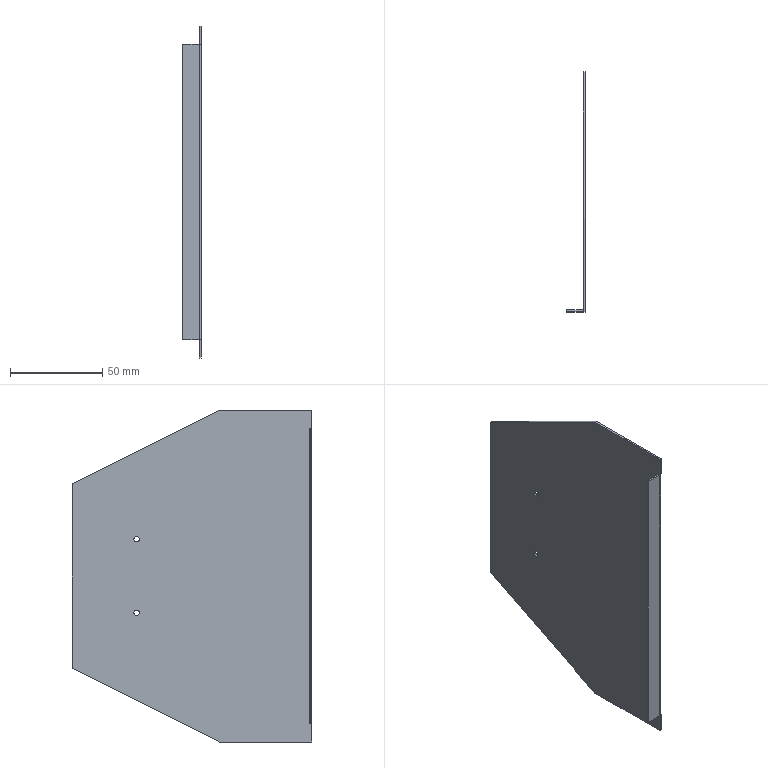Component | SolidWorks | LightBox-1_LightBox2-1 | 1 solid | 24 faces | box 10 x 130 x 180 mm | volume 21585 mm3 | plane 18 | cylinder 6 | commonest cylinder face diameters 3 x4 2.2 x1 0.2 x1
STEP:
#1=CARTESIAN_POINT('',(5.006,-0.2003,2.421));
#2=VERTEX_POINT('',#1);
#3=CARTESIAN_POINT('',(5.006,-0.2003,2.303));
#4=VERTEX_POINT('',#3);
#5=CARTESIAN_POINT('',(5.006,-0.2003,2.362));
#6=DIRECTION('',(1.,0.,0.));
#7=DIRECTION('',(0.,0.,-1.));
#8=AXIS2_PLACEMENT_3D('',#5,#6,#7);
#9=CIRCLE('',#8,0.05906);
#10=EDGE_CURVE('',#2,#4,#9,.T.);
#11=ORIENTED_EDGE('',*,*,#10,.F.);
#12=CARTESIAN_POINT('',(5.045,-0.2003,2.421));
#13=VERTEX_POINT('',#12);
#14=CARTESIAN_POINT('',(5.006,-0.2003,2.421));
#15=DIRECTION('',(1.,0.,0.));
#16=VECTOR('',#15,39.37);
#17=LINE('',#14,#16);
#18=EDGE_CURVE('',#2,#13,#17,.T.);
#19=ORIENTED_EDGE('',*,*,#18,.T.);
#20=CARTESIAN_POINT('',(5.045,-0.2003,2.303));
#21=VERTEX_POINT('',#20);
#22=CARTESIAN_POINT('',(5.045,-0.2003,2.362));
#23=DIRECTION('',(1.,0.,0.));
#24=DIRECTION('',(0.,0.,-1.));
#25=AXIS2_PLACEMENT_3D('',#22,#23,#24);
#26=CIRCLE('',#25,0.05906);
#27=EDGE_CURVE('',#13,#21,#26,.T.);
#28=ORIENTED_EDGE('',*,*,#27,.T.);
#29=CARTESIAN_POINT('',(5.006,-0.2003,2.303));
#30=DIRECTION('',(1.,0.,0.));
#31=VECTOR('',#30,39.37);
#32=LINE('',#29,#31);
#33=EDGE_CURVE('',#4,#21,#32,.T.);
#34=ORIENTED_EDGE('',*,*,#33,.F.);
#35=EDGE_LOOP('',(#11,#19,#28,#34));
#36=FACE_OUTER_BOUND('',#35,.T.);
#37=CARTESIAN_POINT('',(5.006,-0.2003,2.362));
#38=DIRECTION('',(1.,0.,0.));
#39=DIRECTION('',(0.,0.,-1.));
#40=AXIS2_PLACEMENT_3D('',#37,#38,#39);
#41=CYLINDRICAL_SURFACE('',#40,0.05906);
#42=ADVANCED_FACE('',(#36),#41,.F.);
#43=CARTESIAN_POINT('',(5.006,-0.2003,3.996));
#44=VERTEX_POINT('',#43);
#45=CARTESIAN_POINT('',(5.006,-0.2003,3.878));
#46=VERTEX_POINT('',#45);
#47=CARTESIAN_POINT('',(5.006,-0.2003,3.937));
#48=DIRECTION('',(1.,0.,0.));
#49=DIRECTION('',(0.,0.,-1.));
#50=AXIS2_PLACEMENT_3D('',#47,#48,#49);
#51=CIRCLE('',#50,0.05906);
#52=EDGE_CURVE('',#44,#46,#51,.T.);
#53=ORIENTED_EDGE('',*,*,#52,.F.);
#54=CARTESIAN_POINT('',(5.045,-0.2003,3.996));
#55=VERTEX_POINT('',#54);
#56=CARTESIAN_POINT('',(5.006,-0.2003,3.996));
#57=DIRECTION('',(1.,0.,0.));
#58=VECTOR('',#57,39.37);
#59=LINE('',#56,#58);
#60=EDGE_CURVE('',#44,#55,#59,.T.);
#61=ORIENTED_EDGE('',*,*,#60,.T.);
#62=CARTESIAN_POINT('',(5.045,-0.2003,3.878));
#63=VERTEX_POINT('',#62);
#64=CARTESIAN_POINT('',(5.045,-0.2003,3.937));
#65=DIRECTION('',(1.,0.,0.));
#66=DIRECTION('',(0.,0.,-1.));
#67=AXIS2_PLACEMENT_3D('',#64,#65,#66);
#68=CIRCLE('',#67,0.05906);
#69=EDGE_CURVE('',#55,#63,#68,.T.);
#70=ORIENTED_EDGE('',*,*,#69,.T.);
#71=CARTESIAN_POINT('',(5.006,-0.2003,3.878));
#72=DIRECTION('',(1.,0.,0.));
#73=VECTOR('',#72,39.37);
#74=LINE('',#71,#73);
#75=EDGE_CURVE('',#46,#63,#74,.T.);
#76=ORIENTED_EDGE('',*,*,#75,.F.);
#77=EDGE_LOOP('',(#53,#61,#70,#76));
#78=FACE_OUTER_BOUND('',#77,.T.);
#79=CARTESIAN_POINT('',(5.006,-0.2003,3.937));
#80=DIRECTION('',(1.,0.,0.));
#81=DIRECTION('',(0.,0.,-1.));
#82=AXIS2_PLACEMENT_3D('',#79,#80,#81);
#83=CYLINDRICAL_SURFACE('',#82,0.05906);
#84=ADVANCED_FACE('',(#78),#83,.F.);
#85=CARTESIAN_POINT('',(5.006,-3.94,6.299));
#86=VERTEX_POINT('',#85);
#87=CARTESIAN_POINT('',(5.006,-3.94,6.299));
#88=VERTEX_POINT('',#87);
#89=CARTESIAN_POINT('',(5.006,-3.94,6.299));
#90=DIRECTION('',(0.,1.,0.));
#91=VECTOR('',#90,39.37);
#92=LINE('',#89,#91);
#93=EDGE_CURVE('',#86,#88,#92,.T.);
#94=ORIENTED_EDGE('',*,*,#93,.T.);
#95=CARTESIAN_POINT('',(5.045,-3.897,6.299));
#96=VERTEX_POINT('',#95);
#97=CARTESIAN_POINT('',(5.002,-3.897,6.299));
#98=DIRECTION('',(0.,0.,1.));
#99=DIRECTION('',(1.,0.,0.));
#100=AXIS2_PLACEMENT_3D('',#97,#98,#99);
#101=CIRCLE('',#100,0.04331);
#102=EDGE_CURVE('',#88,#96,#101,.T.);
#103=ORIENTED_EDGE('',*,*,#102,.T.);
#104=CARTESIAN_POINT('',(5.045,-3.94,6.299));
#105=VERTEX_POINT('',#104);
#106=CARTESIAN_POINT('',(5.045,-0.9737,6.299));
#107=DIRECTION('',(0.,-1.,0.));
#108=VECTOR('',#107,39.37);
#109=LINE('',#106,#108);
#110=EDGE_CURVE('',#96,#105,#109,.T.);
#111=ORIENTED_EDGE('',*,*,#110,.T.);
#112=CARTESIAN_POINT('',(5.006,-3.94,6.299));
#113=DIRECTION('',(1.,0.,0.));
#114=VECTOR('',#113,39.37);
#115=LINE('',#112,#114);
#116=EDGE_CURVE('',#86,#105,#115,.T.);
#117=ORIENTED_EDGE('',*,*,#116,.F.);
#118=EDGE_LOOP('',(#94,#103,#111,#117));
#119=FACE_OUTER_BOUND('',#118,.T.);
#120=CARTESIAN_POINT('',(5.006,-3.94,6.299));
#121=DIRECTION('',(0.,-0.,-1.));
#122=DIRECTION('',(-1.,0.,-0.));
#123=AXIS2_PLACEMENT_3D('',#120,#121,#122);
#124=PLANE('',#123);
#125=ADVANCED_FACE('',(#119),#124,.T.);
#126=CARTESIAN_POINT('',(5.045,-3.94,0.));
#127=VERTEX_POINT('',#126);
#128=CARTESIAN_POINT('',(5.045,-3.897,0.));
#129=VERTEX_POINT('',#128);
#130=CARTESIAN_POINT('',(5.045,-0.9737,0.));
#131=DIRECTION('',(0.,1.,0.));
#132=VECTOR('',#131,39.37);
#133=LINE('',#130,#132);
#134=EDGE_CURVE('',#127,#129,#133,.T.);
#135=ORIENTED_EDGE('',*,*,#134,.T.);
#136=CARTESIAN_POINT('',(5.006,-3.94,0.));
#137=VERTEX_POINT('',#136);
#138=CARTESIAN_POINT('',(5.002,-3.897,0.));
#139=DIRECTION('',(-0.,0.,-1.));
#140=DIRECTION('',(1.,0.,-0.));
#141=AXIS2_PLACEMENT_3D('',#138,#139,#140);
#142=CIRCLE('',#141,0.04331);
#143=EDGE_CURVE('',#129,#137,#142,.T.);
#144=ORIENTED_EDGE('',*,*,#143,.T.);
#145=CARTESIAN_POINT('',(5.006,-3.94,0.));
#146=VERTEX_POINT('',#145);
#147=CARTESIAN_POINT('',(5.006,-3.897,0.));
#148=DIRECTION('',(0.,-1.,0.));
#149=VECTOR('',#148,39.37);
#150=LINE('',#147,#149);
#151=EDGE_CURVE('',#137,#146,#150,.T.);
#152=ORIENTED_EDGE('',*,*,#151,.T.);
#153=CARTESIAN_POINT('',(5.006,-3.94,0.));
#154=DIRECTION('',(1.,0.,0.));
#155=VECTOR('',#154,39.37);
#156=LINE('',#153,#155);
#157=EDGE_CURVE('',#146,#127,#156,.T.);
#158=ORIENTED_EDGE('',*,*,#157,.T.);
#159=EDGE_LOOP('',(#135,#144,#152,#158));
#160=FACE_OUTER_BOUND('',#159,.T.);
#161=CARTESIAN_POINT('',(5.006,-3.897,0.));
#162=DIRECTION('',(-0.,-0.,1.));
#163=DIRECTION('',(1.,0.,0.));
#164=AXIS2_PLACEMENT_3D('',#161,#162,#163);
#165=PLANE('',#164);
#166=ADVANCED_FACE('',(#160),#165,.T.);
#167=CARTESIAN_POINT('',(5.006,-3.94,6.693));
#168=VERTEX_POINT('',#167);
#169=CARTESIAN_POINT('',(5.006,-3.94,-0.3937));
#170=DIRECTION('',(0.,0.,-1.));
#171=VECTOR('',#170,39.37);
#172=LINE('',#169,#171);
#173=EDGE_CURVE('',#168,#86,#172,.T.);
#174=ORIENTED_EDGE('',*,*,#173,.T.);
#175=ORIENTED_EDGE('',*,*,#116,.T.);
#176=CARTESIAN_POINT('',(5.045,-3.94,6.693));
#177=VERTEX_POINT('',#176);
#178=CARTESIAN_POINT('',(5.045,-3.94,-0.3937));
#179=DIRECTION('',(0.,0.,-1.));
#180=VECTOR('',#179,39.37);
#181=LINE('',#178,#180);
#182=EDGE_CURVE('',#177,#105,#181,.T.);
#183=ORIENTED_EDGE('',*,*,#182,.F.);
#184=CARTESIAN_POINT('',(5.006,-3.94,6.693));
#185=DIRECTION('',(1.,0.,0.));
#186=VECTOR('',#185,39.37);
#187=LINE('',#184,#186);
#188=EDGE_CURVE('',#168,#177,#187,.T.);
#189=ORIENTED_EDGE('',*,*,#188,.F.);
#190=EDGE_LOOP('',(#174,#175,#183,#189));
#191=FACE_OUTER_BOUND('',#190,.T.);
#192=CARTESIAN_POINT('',(5.006,-3.94,-0.3937));
#193=DIRECTION('',(0.,-1.,-0.));
#194=DIRECTION('',(0.,0.,-1.));
#195=AXIS2_PLACEMENT_3D('',#192,#193,#194);
#196=PLANE('',#195);
#197=ADVANCED_FACE('',(#191),#196,.T.);
#198=CARTESIAN_POINT('',(5.045,-3.94,-0.3937));
#199=VERTEX_POINT('',#198);
#200=CARTESIAN_POINT('',(5.045,-3.94,-0.3937));
#201=DIRECTION('',(0.,0.,-1.));
#202=VECTOR('',#201,39.37);
#203=LINE('',#200,#202);
#204=EDGE_CURVE('',#127,#199,#203,.T.);
#205=ORIENTED_EDGE('',*,*,#204,.F.);
#206=ORIENTED_EDGE('',*,*,#157,.F.);
#207=CARTESIAN_POINT('',(5.006,-3.94,-0.3937));
#208=VERTEX_POINT('',#207);
#209=CARTESIAN_POINT('',(5.006,-3.94,-0.3937));
#210=DIRECTION('',(0.,0.,-1.));
#211=VECTOR('',#210,39.37);
#212=LINE('',#209,#211);
#213=EDGE_CURVE('',#146,#208,#212,.T.);
#214=ORIENTED_EDGE('',*,*,#213,.T.);
#215=CARTESIAN_POINT('',(5.006,-3.94,-0.3937));
#216=DIRECTION('',(1.,0.,0.));
#217=VECTOR('',#216,39.37);
#218=LINE('',#215,#217);
#219=EDGE_CURVE('',#208,#199,#218,.T.);
#220=ORIENTED_EDGE('',*,*,#219,.T.);
#221=EDGE_LOOP('',(#205,#206,#214,#220));
#222=FACE_OUTER_BOUND('',#221,.T.);
#223=CARTESIAN_POINT('',(5.006,-3.94,-0.3937));
#224=DIRECTION('',(0.,-1.,-0.));
#225=DIRECTION('',(0.,0.,-1.));
#226=AXIS2_PLACEMENT_3D('',#223,#224,#225);
#227=PLANE('',#226);
#228=ADVANCED_FACE('',(#222),#227,.T.);
#229=CARTESIAN_POINT('',(5.006,-0.2003,2.362));
#230=DIRECTION('',(1.,0.,0.));
#231=DIRECTION('',(0.,0.,-1.));
#232=AXIS2_PLACEMENT_3D('',#229,#230,#231);
#233=CIRCLE('',#232,0.05906);
#234=EDGE_CURVE('',#4,#2,#233,.T.);
#235=ORIENTED_EDGE('',*,*,#234,.T.);
#236=ORIENTED_EDGE('',*,*,#10,.T.);
#237=EDGE_LOOP('',(#235,#236));
#238=FACE_BOUND('',#237,.T.);
#239=CARTESIAN_POINT('',(5.006,-0.2003,3.937));
#240=DIRECTION('',(1.,0.,0.));
#241=DIRECTION('',(0.,0.,-1.));
#242=AXIS2_PLACEMENT_3D('',#239,#240,#241);
#243=CIRCLE('',#242,0.05906);
#244=EDGE_CURVE('',#46,#44,#243,.T.);
#245=ORIENTED_EDGE('',*,*,#244,.T.);
#246=ORIENTED_EDGE('',*,*,#52,.T.);
#247=EDGE_LOOP('',(#245,#246));
#248=FACE_BOUND('',#247,.T.);
#249=CARTESIAN_POINT('',(5.006,-3.897,6.299));
#250=VERTEX_POINT('',#249);
#251=CARTESIAN_POINT('',(5.006,-3.897,0.));
#252=VERTEX_POINT('',#251);
#253=CARTESIAN_POINT('',(5.006,-3.897,6.299));
#254=DIRECTION('',(-0.,0.,-1.));
#255=VECTOR('',#254,39.37);
#256=LINE('',#253,#255);
#257=EDGE_CURVE('',#250,#252,#256,.T.);
#258=ORIENTED_EDGE('',*,*,#257,.F.);
#259=CARTESIAN_POINT('',(5.006,-3.94,6.299));
#260=DIRECTION('',(0.,1.,0.));
#261=VECTOR('',#260,39.37);
#262=LINE('',#259,#261);
#263=EDGE_CURVE('',#88,#250,#262,.T.);
#264=ORIENTED_EDGE('',*,*,#263,.F.);
#265=ORIENTED_EDGE('',*,*,#93,.F.);
#266=ORIENTED_EDGE('',*,*,#173,.F.);
#267=CARTESIAN_POINT('',(5.006,-1.972,6.693));
#268=VERTEX_POINT('',#267);
#269=CARTESIAN_POINT('',(5.006,-3.94,6.693));
#270=DIRECTION('',(0.,-1.,0.));
#271=VECTOR('',#270,39.37);
#272=LINE('',#269,#271);
#273=EDGE_CURVE('',#268,#168,#272,.T.);
#274=ORIENTED_EDGE('',*,*,#273,.F.);
#275=CARTESIAN_POINT('',(5.006,1.178,5.118));
#276=VERTEX_POINT('',#275);
#277=CARTESIAN_POINT('',(5.006,-1.972,6.693));
#278=DIRECTION('',(0.,-0.8944,0.4472));
#279=VECTOR('',#278,39.37);
#280=LINE('',#277,#279);
#281=EDGE_CURVE('',#276,#268,#280,.T.);
#282=ORIENTED_EDGE('',*,*,#281,.F.);
#283=CARTESIAN_POINT('',(5.006,1.178,1.181));
#284=VERTEX_POINT('',#283);
#285=CARTESIAN_POINT('',(5.006,1.178,5.118));
#286=DIRECTION('',(0.,0.,1.));
#287=VECTOR('',#286,39.37);
#288=LINE('',#285,#287);
#289=EDGE_CURVE('',#284,#276,#288,.T.);
#290=ORIENTED_EDGE('',*,*,#289,.F.);
#291=CARTESIAN_POINT('',(5.006,-1.972,-0.3937));
#292=VERTEX_POINT('',#291);
#293=CARTESIAN_POINT('',(5.006,1.178,1.181));
#294=DIRECTION('',(0.,0.8944,0.4472));
#295=VECTOR('',#294,39.37);
#296=LINE('',#293,#295);
#297=EDGE_CURVE('',#292,#284,#296,.T.);
#298=ORIENTED_EDGE('',*,*,#297,.F.);
#299=CARTESIAN_POINT('',(5.006,-1.972,-0.3937));
#300=DIRECTION('',(0.,1.,0.));
#301=VECTOR('',#300,39.37);
#302=LINE('',#299,#301);
#303=EDGE_CURVE('',#208,#292,#302,.T.);
#304=ORIENTED_EDGE('',*,*,#303,.F.);
#305=ORIENTED_EDGE('',*,*,#213,.F.);
#306=ORIENTED_EDGE('',*,*,#151,.F.);
#307=CARTESIAN_POINT('',(5.006,-3.897,0.));
#308=DIRECTION('',(0.,-1.,0.));
#309=VECTOR('',#308,39.37);
#310=LINE('',#307,#309);
#311=EDGE_CURVE('',#252,#137,#310,.T.);
#312=ORIENTED_EDGE('',*,*,#311,.F.);
#313=EDGE_LOOP('',(#258,#264,#265,#266,#274,#282,#290,#298,#304,#305,#306,#312));
#314=FACE_OUTER_BOUND('',#313,.T.);
#315=CARTESIAN_POINT('',(5.006,-0.9737,3.033));
#316=DIRECTION('',(-1.,0.,0.));
#317=DIRECTION('',(0.,0.,1.));
#318=AXIS2_PLACEMENT_3D('',#315,#316,#317);
#319=PLANE('',#318);
#320=ADVANCED_FACE('',(#238,#248,#314),#319,.T.);
#321=CARTESIAN_POINT('',(5.045,-0.2003,3.937));
#322=DIRECTION('',(1.,0.,0.));
#323=DIRECTION('',(0.,0.,-1.));
#324=AXIS2_PLACEMENT_3D('',#321,#322,#323);
#325=CIRCLE('',#324,0.05906);
#326=EDGE_CURVE('',#63,#55,#325,.T.);
#327=ORIENTED_EDGE('',*,*,#326,.F.);
#328=ORIENTED_EDGE('',*,*,#69,.F.);
#329=EDGE_LOOP('',(#327,#328));
#330=FACE_BOUND('',#329,.T.);
#331=CARTESIAN_POINT('',(5.045,-0.2003,2.362));
#332=DIRECTION('',(1.,0.,0.));
#333=DIRECTION('',(0.,0.,-1.));
#334=AXIS2_PLACEMENT_3D('',#331,#332,#333);
#335=CIRCLE('',#334,0.05906);
#336=EDGE_CURVE('',#21,#13,#335,.T.);
#337=ORIENTED_EDGE('',*,*,#336,.F.);
#338=ORIENTED_EDGE('',*,*,#27,.F.);
#339=EDGE_LOOP('',(#337,#338));
#340=FACE_BOUND('',#339,.T.);
#341=ORIENTED_EDGE('',*,*,#110,.F.);
#342=CARTESIAN_POINT('',(5.045,-3.897,6.299));
#343=DIRECTION('',(-0.,0.,-1.));
#344=VECTOR('',#343,39.37);
#345=LINE('',#342,#344);
#346=EDGE_CURVE('',#96,#129,#345,.T.);
#347=ORIENTED_EDGE('',*,*,#346,.T.);
#348=ORIENTED_EDGE('',*,*,#134,.F.);
#349=ORIENTED_EDGE('',*,*,#204,.T.);
#350=CARTESIAN_POINT('',(5.045,-1.972,-0.3937));
#351=VERTEX_POINT('',#350);
#352=CARTESIAN_POINT('',(5.045,-1.972,-0.3937));
#353=DIRECTION('',(0.,1.,0.));
#354=VECTOR('',#353,39.37);
#355=LINE('',#352,#354);
#356=EDGE_CURVE('',#199,#351,#355,.T.);
#357=ORIENTED_EDGE('',*,*,#356,.T.);
#358=CARTESIAN_POINT('',(5.045,1.178,1.181));
#359=VERTEX_POINT('',#358);
#360=CARTESIAN_POINT('',(5.045,1.178,1.181));
#361=DIRECTION('',(0.,0.8944,0.4472));
#362=VECTOR('',#361,39.37);
#363=LINE('',#360,#362);
#364=EDGE_CURVE('',#351,#359,#363,.T.);
#365=ORIENTED_EDGE('',*,*,#364,.T.);
#366=CARTESIAN_POINT('',(5.045,1.178,5.118));
#367=VERTEX_POINT('',#366);
#368=CARTESIAN_POINT('',(5.045,1.178,5.118));
#369=DIRECTION('',(0.,0.,1.));
#370=VECTOR('',#369,39.37);
#371=LINE('',#368,#370);
#372=EDGE_CURVE('',#359,#367,#371,.T.);
#373=ORIENTED_EDGE('',*,*,#372,.T.);
#374=CARTESIAN_POINT('',(5.045,-1.972,6.693));
#375=VERTEX_POINT('',#374);
#376=CARTESIAN_POINT('',(5.045,-1.972,6.693));
#377=DIRECTION('',(0.,-0.8944,0.4472));
#378=VECTOR('',#377,39.37);
#379=LINE('',#376,#378);
#380=EDGE_CURVE('',#367,#375,#379,.T.);
#381=ORIENTED_EDGE('',*,*,#380,.T.);
#382=CARTESIAN_POINT('',(5.045,-3.94,6.693));
#383=DIRECTION('',(0.,-1.,0.));
#384=VECTOR('',#383,39.37);
#385=LINE('',#382,#384);
#386=EDGE_CURVE('',#375,#177,#385,.T.);
#387=ORIENTED_EDGE('',*,*,#386,.T.);
#388=ORIENTED_EDGE('',*,*,#182,.T.);
#389=EDGE_LOOP('',(#341,#347,#348,#349,#357,#365,#373,#381,#387,#388));
#390=FACE_OUTER_BOUND('',#389,.T.);
#391=CARTESIAN_POINT('',(5.045,-0.9737,3.033));
#392=DIRECTION('',(-1.,0.,0.));
#393=DIRECTION('',(0.,0.,1.));
#394=AXIS2_PLACEMENT_3D('',#391,#392,#393);
#395=PLANE('',#394);
#396=ADVANCED_FACE('',(#330,#340,#390),#395,.F.);
#397=ORIENTED_EDGE('',*,*,#380,.F.);
#398=CARTESIAN_POINT('',(5.006,1.178,5.118));
#399=DIRECTION('',(1.,0.,0.));
#400=VECTOR('',#399,39.37);
#401=LINE('',#398,#400);
#402=EDGE_CURVE('',#276,#367,#401,.T.);
#403=ORIENTED_EDGE('',*,*,#402,.F.);
#404=ORIENTED_EDGE('',*,*,#281,.T.);
#405=CARTESIAN_POINT('',(5.006,-1.972,6.693));
#406=DIRECTION('',(1.,0.,0.));
#407=VECTOR('',#406,39.37);
#408=LINE('',#405,#407);
#409=EDGE_CURVE('',#268,#375,#408,.T.);
#410=ORIENTED_EDGE('',*,*,#409,.T.);
#411=EDGE_LOOP('',(#397,#403,#404,#410));
#412=FACE_OUTER_BOUND('',#411,.T.);
#413=CARTESIAN_POINT('',(5.006,-1.972,6.693));
#414=DIRECTION('',(0.,0.4472,0.8944));
#415=DIRECTION('',(0.,-0.8944,0.4472));
#416=AXIS2_PLACEMENT_3D('',#413,#414,#415);
#417=PLANE('',#416);
#418=ADVANCED_FACE('',(#412),#417,.T.);
#419=ORIENTED_EDGE('',*,*,#372,.F.);
#420=CARTESIAN_POINT('',(5.006,1.178,1.181));
#421=DIRECTION('',(1.,0.,0.));
#422=VECTOR('',#421,39.37);
#423=LINE('',#420,#422);
#424=EDGE_CURVE('',#284,#359,#423,.T.);
#425=ORIENTED_EDGE('',*,*,#424,.F.);
#426=ORIENTED_EDGE('',*,*,#289,.T.);
#427=ORIENTED_EDGE('',*,*,#402,.T.);
#428=EDGE_LOOP('',(#419,#425,#426,#427));
#429=FACE_OUTER_BOUND('',#428,.T.);
#430=CARTESIAN_POINT('',(5.006,1.178,5.118));
#431=DIRECTION('',(0.,1.,0.));
#432=DIRECTION('',(0.,0.,1.));
#433=AXIS2_PLACEMENT_3D('',#430,#431,#432);
#434=PLANE('',#433);
#435=ADVANCED_FACE('',(#429),#434,.T.);
#436=ORIENTED_EDGE('',*,*,#364,.F.);
#437=CARTESIAN_POINT('',(5.006,-1.972,-0.3937));
#438=DIRECTION('',(1.,0.,0.));
#439=VECTOR('',#438,39.37);
#440=LINE('',#437,#439);
#441=EDGE_CURVE('',#292,#351,#440,.T.);
#442=ORIENTED_EDGE('',*,*,#441,.F.);
#443=ORIENTED_EDGE('',*,*,#297,.T.);
#444=ORIENTED_EDGE('',*,*,#424,.T.);
#445=EDGE_LOOP('',(#436,#442,#443,#444));
#446=FACE_OUTER_BOUND('',#445,.T.);
#447=CARTESIAN_POINT('',(5.006,1.178,1.181));
#448=DIRECTION('',(0.,0.4472,-0.8944));
#449=DIRECTION('',(0.,0.8944,0.4472));
#450=AXIS2_PLACEMENT_3D('',#447,#448,#449);
#451=PLANE('',#450);
#452=ADVANCED_FACE('',(#446),#451,.T.);
#453=ORIENTED_EDGE('',*,*,#356,.F.);
#454=ORIENTED_EDGE('',*,*,#219,.F.);
#455=ORIENTED_EDGE('',*,*,#303,.T.);
#456=ORIENTED_EDGE('',*,*,#441,.T.);
#457=EDGE_LOOP('',(#453,#454,#455,#456));
#458=FACE_OUTER_BOUND('',#457,.T.);
#459=CARTESIAN_POINT('',(5.006,-1.972,-0.3937));
#460=DIRECTION('',(0.,0.,-1.));
#461=DIRECTION('',(0.,1.,0.));
#462=AXIS2_PLACEMENT_3D('',#459,#460,#461);
#463=PLANE('',#462);
#464=ADVANCED_FACE('',(#458),#463,.T.);
#465=ORIENTED_EDGE('',*,*,#386,.F.);
#466=ORIENTED_EDGE('',*,*,#409,.F.);
#467=ORIENTED_EDGE('',*,*,#273,.T.);
#468=ORIENTED_EDGE('',*,*,#188,.T.);
#469=EDGE_LOOP('',(#465,#466,#467,#468));
#470=FACE_OUTER_BOUND('',#469,.T.);
#471=CARTESIAN_POINT('',(5.006,-3.94,6.693));
#472=DIRECTION('',(0.,0.,1.));
#473=DIRECTION('',(1.,0.,0.));
#474=AXIS2_PLACEMENT_3D('',#471,#472,#473);
#475=PLANE('',#474);
#476=ADVANCED_FACE('',(#470),#475,.T.);
#477=ORIENTED_EDGE('',*,*,#60,.F.);
#478=ORIENTED_EDGE('',*,*,#244,.F.);
#479=ORIENTED_EDGE('',*,*,#75,.T.);
#480=ORIENTED_EDGE('',*,*,#326,.T.);
#481=EDGE_LOOP('',(#477,#478,#479,#480));
#482=FACE_OUTER_BOUND('',#481,.T.);
#483=CARTESIAN_POINT('',(5.006,-0.2003,3.937));
#484=DIRECTION('',(1.,0.,0.));
#485=DIRECTION('',(0.,0.,-1.));
#486=AXIS2_PLACEMENT_3D('',#483,#484,#485);
#487=CYLINDRICAL_SURFACE('',#486,0.05906);
#488=ADVANCED_FACE('',(#482),#487,.F.);
#489=ORIENTED_EDGE('',*,*,#18,.F.);
#490=ORIENTED_EDGE('',*,*,#234,.F.);
#491=ORIENTED_EDGE('',*,*,#33,.T.);
#492=ORIENTED_EDGE('',*,*,#336,.T.);
#493=EDGE_LOOP('',(#489,#490,#491,#492));
#494=FACE_OUTER_BOUND('',#493,.T.);
#495=CARTESIAN_POINT('',(5.006,-0.2003,2.362));
#496=DIRECTION('',(1.,0.,0.));
#497=DIRECTION('',(0.,0.,-1.));
#498=AXIS2_PLACEMENT_3D('',#495,#496,#497);
#499=CYLINDRICAL_SURFACE('',#498,0.05906);
#500=ADVANCED_FACE('',(#494),#499,.F.);
#501=CARTESIAN_POINT('',(5.002,-3.901,0.));
#502=VERTEX_POINT('',#501);
#503=CARTESIAN_POINT('',(5.002,-3.897,0.));
#504=DIRECTION('',(-0.,0.,-1.));
#505=DIRECTION('',(1.,0.,-0.));
#506=AXIS2_PLACEMENT_3D('',#503,#504,#505);
#507=CIRCLE('',#506,0.003937);
#508=EDGE_CURVE('',#252,#502,#507,.T.);
#509=ORIENTED_EDGE('',*,*,#508,.F.);
#510=ORIENTED_EDGE('',*,*,#311,.T.);
#511=CARTESIAN_POINT('',(5.002,-3.94,0.));
#512=VERTEX_POINT('',#511);
#513=CARTESIAN_POINT('',(5.002,-3.897,0.));
#514=DIRECTION('',(-0.,0.,-1.));
#515=DIRECTION('',(1.,0.,-0.));
#516=AXIS2_PLACEMENT_3D('',#513,#514,#515);
#517=CIRCLE('',#516,0.04331);
#518=EDGE_CURVE('',#137,#512,#517,.T.);
#519=ORIENTED_EDGE('',*,*,#518,.T.);
#520=CARTESIAN_POINT('',(5.002,-3.94,0.));
#521=DIRECTION('',(0.,-1.,-0.));
#522=VECTOR('',#521,39.37);
#523=LINE('',#520,#522);
#524=EDGE_CURVE('',#502,#512,#523,.T.);
#525=ORIENTED_EDGE('',*,*,#524,.F.);
#526=EDGE_LOOP('',(#509,#510,#519,#525));
#527=FACE_OUTER_BOUND('',#526,.T.);
#528=CARTESIAN_POINT('',(5.002,-3.897,0.));
#529=DIRECTION('',(-0.,0.,-1.));
#530=DIRECTION('',(-1.,0.,0.));
#531=AXIS2_PLACEMENT_3D('',#528,#529,#530);
#532=PLANE('',#531);
#533=ADVANCED_FACE('',(#527),#532,.T.);
#534=CARTESIAN_POINT('',(5.002,-3.94,6.299));
#535=VERTEX_POINT('',#534);
#536=CARTESIAN_POINT('',(5.002,-3.897,6.299));
#537=DIRECTION('',(0.,0.,1.));
#538=DIRECTION('',(1.,0.,0.));
#539=AXIS2_PLACEMENT_3D('',#536,#537,#538);
#540=CIRCLE('',#539,0.04331);
#541=EDGE_CURVE('',#535,#88,#540,.T.);
#542=ORIENTED_EDGE('',*,*,#541,.T.);
#543=ORIENTED_EDGE('',*,*,#263,.T.);
#544=CARTESIAN_POINT('',(5.002,-3.901,6.299));
#545=VERTEX_POINT('',#544);
#546=CARTESIAN_POINT('',(5.002,-3.897,6.299));
#547=DIRECTION('',(0.,0.,1.));
#548=DIRECTION('',(1.,0.,0.));
#549=AXIS2_PLACEMENT_3D('',#546,#547,#548);
#550=CIRCLE('',#549,0.003937);
#551=EDGE_CURVE('',#545,#250,#550,.T.);
#552=ORIENTED_EDGE('',*,*,#551,.F.);
#553=CARTESIAN_POINT('',(5.002,-3.901,6.299));
#554=DIRECTION('',(0.,-1.,-0.));
#555=VECTOR('',#554,39.37);
#556=LINE('',#553,#555);
#557=EDGE_CURVE('',#545,#535,#556,.T.);
#558=ORIENTED_EDGE('',*,*,#557,.T.);
#559=EDGE_LOOP('',(#542,#543,#552,#558));
#560=FACE_OUTER_BOUND('',#559,.T.);
#561=CARTESIAN_POINT('',(5.002,-3.897,6.299));
#562=DIRECTION('',(-0.,0.,-1.));
#563=DIRECTION('',(-1.,0.,0.));
#564=AXIS2_PLACEMENT_3D('',#561,#562,#563);
#565=PLANE('',#564);
#566=ADVANCED_FACE('',(#560),#565,.F.);
#567=ORIENTED_EDGE('',*,*,#346,.F.);
#568=ORIENTED_EDGE('',*,*,#102,.F.);
#569=ORIENTED_EDGE('',*,*,#541,.F.);
#570=CARTESIAN_POINT('',(5.002,-3.94,3.033));
#571=DIRECTION('',(0.,-0.,1.));
#572=VECTOR('',#571,39.37);
#573=LINE('',#570,#572);
#574=EDGE_CURVE('',#512,#535,#573,.T.);
#575=ORIENTED_EDGE('',*,*,#574,.F.);
#576=ORIENTED_EDGE('',*,*,#518,.F.);
#577=ORIENTED_EDGE('',*,*,#143,.F.);
#578=EDGE_LOOP('',(#567,#568,#569,#575,#576,#577));
#579=FACE_OUTER_BOUND('',#578,.T.);
#580=CARTESIAN_POINT('',(5.002,-3.897,6.299));
#581=DIRECTION('',(0.,0.,1.));
#582=DIRECTION('',(0.,-1.,0.));
#583=AXIS2_PLACEMENT_3D('',#580,#581,#582);
#584=CYLINDRICAL_SURFACE('',#583,0.04331);
#585=ADVANCED_FACE('',(#579),#584,.T.);
#586=ORIENTED_EDGE('',*,*,#257,.T.);
#587=ORIENTED_EDGE('',*,*,#508,.T.);
#588=CARTESIAN_POINT('',(5.002,-3.901,0.));
#589=DIRECTION('',(0.,-0.,1.));
#590=VECTOR('',#589,39.37);
#591=LINE('',#588,#590);
#592=EDGE_CURVE('',#502,#545,#591,.T.);
#593=ORIENTED_EDGE('',*,*,#592,.T.);
#594=ORIENTED_EDGE('',*,*,#551,.T.);
#595=EDGE_LOOP('',(#586,#587,#593,#594));
#596=FACE_OUTER_BOUND('',#595,.T.);
#597=CARTESIAN_POINT('',(5.002,-3.897,6.299));
#598=DIRECTION('',(0.,0.,1.));
#599=DIRECTION('',(0.,-1.,0.));
#600=AXIS2_PLACEMENT_3D('',#597,#598,#599);
#601=CYLINDRICAL_SURFACE('',#600,0.003937);
#602=ADVANCED_FACE('',(#596),#601,.F.);
#603=CARTESIAN_POINT('',(4.651,-3.94,6.299));
#604=VERTEX_POINT('',#603);
#605=CARTESIAN_POINT('',(5.006,-3.94,6.299));
#606=DIRECTION('',(1.,0.,0.));
#607=VECTOR('',#606,39.37);
#608=LINE('',#605,#607);
#609=EDGE_CURVE('',#604,#535,#608,.T.);
#610=ORIENTED_EDGE('',*,*,#609,.T.);
#611=ORIENTED_EDGE('',*,*,#557,.F.);
#612=CARTESIAN_POINT('',(4.651,-3.901,6.299));
#613=VERTEX_POINT('',#612);
#614=CARTESIAN_POINT('',(5.045,-3.901,6.299));
#615=DIRECTION('',(1.,0.,0.));
#616=VECTOR('',#615,39.37);
#617=LINE('',#614,#616);
#618=EDGE_CURVE('',#613,#545,#617,.T.);
#619=ORIENTED_EDGE('',*,*,#618,.F.);
#620=CARTESIAN_POINT('',(4.651,-3.94,6.299));
#621=DIRECTION('',(-0.,1.,0.));
#622=VECTOR('',#621,39.37);
#623=LINE('',#620,#622);
#624=EDGE_CURVE('',#604,#613,#623,.T.);
#625=ORIENTED_EDGE('',*,*,#624,.F.);
#626=EDGE_LOOP('',(#610,#611,#619,#625));
#627=FACE_OUTER_BOUND('',#626,.T.);
#628=CARTESIAN_POINT('',(5.006,-3.94,6.299));
#629=DIRECTION('',(0.,-0.,1.));
#630=DIRECTION('',(0.,-1.,-0.));
#631=AXIS2_PLACEMENT_3D('',#628,#629,#630);
#632=PLANE('',#631);
#633=ADVANCED_FACE('',(#627),#632,.T.);
#634=CARTESIAN_POINT('',(4.651,-3.901,0.));
#635=VERTEX_POINT('',#634);
#636=CARTESIAN_POINT('',(5.045,-3.901,0.));
#637=DIRECTION('',(-1.,-0.,0.));
#638=VECTOR('',#637,39.37);
#639=LINE('',#636,#638);
#640=EDGE_CURVE('',#502,#635,#639,.T.);
#641=ORIENTED_EDGE('',*,*,#640,.F.);
#642=ORIENTED_EDGE('',*,*,#524,.T.);
#643=CARTESIAN_POINT('',(4.651,-3.94,0.));
#644=VERTEX_POINT('',#643);
#645=CARTESIAN_POINT('',(4.651,-3.94,0.));
#646=DIRECTION('',(-1.,-0.,0.));
#647=VECTOR('',#646,39.37);
#648=LINE('',#645,#647);
#649=EDGE_CURVE('',#512,#644,#648,.T.);
#650=ORIENTED_EDGE('',*,*,#649,.T.);
#651=CARTESIAN_POINT('',(4.651,-3.94,0.));
#652=DIRECTION('',(-0.,1.,0.));
#653=VECTOR('',#652,39.37);
#654=LINE('',#651,#653);
#655=EDGE_CURVE('',#644,#635,#654,.T.);
#656=ORIENTED_EDGE('',*,*,#655,.T.);
#657=EDGE_LOOP('',(#641,#642,#650,#656));
#658=FACE_OUTER_BOUND('',#657,.T.);
#659=CARTESIAN_POINT('',(4.651,-3.94,0.));
#660=DIRECTION('',(-0.,0.,-1.));
#661=DIRECTION('',(0.,1.,0.));
#662=AXIS2_PLACEMENT_3D('',#659,#660,#661);
#663=PLANE('',#662);
#664=ADVANCED_FACE('',(#658),#663,.T.);
#665=ORIENTED_EDGE('',*,*,#649,.F.);
#666=ORIENTED_EDGE('',*,*,#574,.T.);
#667=ORIENTED_EDGE('',*,*,#609,.F.);
#668=CARTESIAN_POINT('',(4.651,-3.94,6.299));
#669=DIRECTION('',(0.,-0.,1.));
#670=VECTOR('',#669,39.37);
#671=LINE('',#668,#670);
#672=EDGE_CURVE('',#644,#604,#671,.T.);
#673=ORIENTED_EDGE('',*,*,#672,.F.);
#674=EDGE_LOOP('',(#665,#666,#667,#673));
#675=FACE_OUTER_BOUND('',#674,.T.);
#676=CARTESIAN_POINT('',(5.045,-3.94,3.033));
#677=DIRECTION('',(0.,-1.,-0.));
#678=DIRECTION('',(1.,0.,0.));
#679=AXIS2_PLACEMENT_3D('',#676,#677,#678);
#680=PLANE('',#679);
#681=ADVANCED_FACE('',(#675),#680,.T.);
#682=ORIENTED_EDGE('',*,*,#592,.F.);
#683=ORIENTED_EDGE('',*,*,#640,.T.);
#684=CARTESIAN_POINT('',(4.651,-3.901,3.033));
#685=DIRECTION('',(0.,-0.,1.));
#686=VECTOR('',#685,39.37);
#687=LINE('',#684,#686);
#688=EDGE_CURVE('',#635,#613,#687,.T.);
#689=ORIENTED_EDGE('',*,*,#688,.T.);
#690=ORIENTED_EDGE('',*,*,#618,.T.);
#691=EDGE_LOOP('',(#682,#683,#689,#690));
#692=FACE_OUTER_BOUND('',#691,.T.);
#693=CARTESIAN_POINT('',(5.045,-3.901,3.033));
#694=DIRECTION('',(0.,-1.,-0.));
#695=DIRECTION('',(1.,0.,0.));
#696=AXIS2_PLACEMENT_3D('',#693,#694,#695);
#697=PLANE('',#696);
#698=ADVANCED_FACE('',(#692),#697,.F.);
#699=ORIENTED_EDGE('',*,*,#688,.F.);
#700=ORIENTED_EDGE('',*,*,#655,.F.);
#701=ORIENTED_EDGE('',*,*,#672,.T.);
#702=ORIENTED_EDGE('',*,*,#624,.T.);
#703=EDGE_LOOP('',(#699,#700,#701,#702));
#704=FACE_OUTER_BOUND('',#703,.T.);
#705=CARTESIAN_POINT('',(4.651,-3.94,6.299));
#706=DIRECTION('',(-1.,-0.,-0.));
#707=DIRECTION('',(0.,-1.,0.));
#708=AXIS2_PLACEMENT_3D('',#705,#706,#707);
#709=PLANE('',#708);
#710=ADVANCED_FACE('',(#704),#709,.T.);
#711=CLOSED_SHELL('',(#42,#84,#125,#166,#197,#228,#320,#396,#418,#435,#452,#464,#476,#488,#500,#533,#566,#585,#602,#633,#664,#681,#698,#710));
#712=MANIFOLD_SOLID_BREP('',#711);
#713=CARTESIAN_POINT('',(0.,0.,0.));
#714=DIRECTION('',(0.,0.,1.));
#715=DIRECTION('',(1.,0.,0.));
#716=AXIS2_PLACEMENT_3D('',#713,#714,#715);
#717=(LENGTH_UNIT()NAMED_UNIT(*)SI_UNIT($,.METRE.));
#718=LENGTH_MEASURE_WITH_UNIT(LENGTH_MEASURE(0.0254),#717);
#719=DIMENSIONAL_EXPONENTS(1.,0.,0.,0.,0.,0.,0.);
#720=(CONVERSION_BASED_UNIT('',#718)LENGTH_UNIT()NAMED_UNIT(#719));
#721=UNCERTAINTY_MEASURE_WITH_UNIT(LENGTH_MEASURE(0.00001),#720,'','');
#722=(NAMED_UNIT(*)PLANE_ANGLE_UNIT()SI_UNIT($,.RADIAN.));
#723=(NAMED_UNIT(*)SI_UNIT($,.STERADIAN.)SOLID_ANGLE_UNIT());
#724=(GEOMETRIC_REPRESENTATION_CONTEXT(3)GLOBAL_UNCERTAINTY_ASSIGNED_CONTEXT((#721))GLOBAL_UNIT_ASSIGNED_CONTEXT((#720,#722,#723))REPRESENTATION_CONTEXT('',''));
#725=ADVANCED_BREP_SHAPE_REPRESENTATION('',(#712,#716),#724);
#726=COLOUR_RGB('',0.7922,0.8196,0.9333);
#727=FILL_AREA_STYLE_COLOUR('',#726);
#728=FILL_AREA_STYLE('',(#727));
#729=SURFACE_STYLE_FILL_AREA(#728);
#730=SURFACE_SIDE_STYLE('',(#729));
#731=SURFACE_STYLE_USAGE(.BOTH.,#730);
#732=PRESENTATION_STYLE_ASSIGNMENT((#731));
#733=STYLED_ITEM('',(#732),#712);
#734=PRESENTATION_LAYER_ASSIGNMENT('','',(#733));
#735=(LENGTH_UNIT()NAMED_UNIT(*)SI_UNIT($,.METRE.));
#736=LENGTH_MEASURE_WITH_UNIT(LENGTH_MEASURE(0.0254),#735);
#737=DIMENSIONAL_EXPONENTS(1.,0.,0.,0.,0.,0.,0.);
#738=(CONVERSION_BASED_UNIT('',#736)LENGTH_UNIT()NAMED_UNIT(#737));
#739=UNCERTAINTY_MEASURE_WITH_UNIT(LENGTH_MEASURE(0.00001),#738,'','');
#740=(NAMED_UNIT(*)PLANE_ANGLE_UNIT()SI_UNIT($,.RADIAN.));
#741=(NAMED_UNIT(*)SI_UNIT($,.STERADIAN.)SOLID_ANGLE_UNIT());
#742=(GEOMETRIC_REPRESENTATION_CONTEXT(3)GLOBAL_UNCERTAINTY_ASSIGNED_CONTEXT((#739))GLOBAL_UNIT_ASSIGNED_CONTEXT((#738,#740,#741))REPRESENTATION_CONTEXT('',''));
#743=MECHANICAL_DESIGN_GEOMETRIC_PRESENTATION_REPRESENTATION('',(#733),#742);